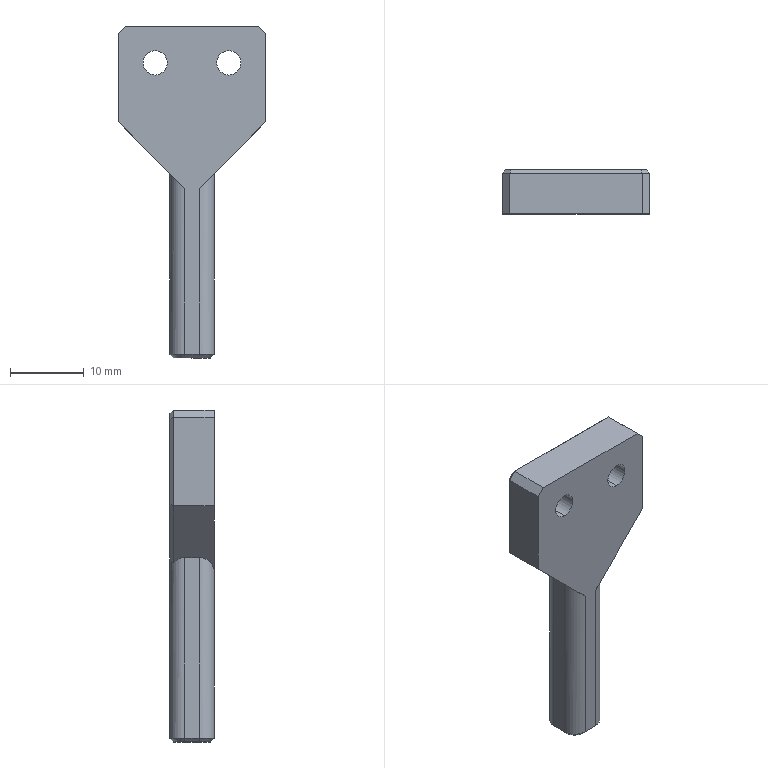Component | SolidWorks | GripperJaw3-1 | 1 solid | 35 faces | box 20 x 6 x 45 mm | volume 2802 mm3 | plane 23 | cylinder 8 | cone 4 | commonest cylinder face diameters 3.3 x4 4 x4
STEP:
#1=COLOUR_RGB('',0.7922,0.8196,0.9333);
#2=FILL_AREA_STYLE_COLOUR('',#1);
#3=FILL_AREA_STYLE('',(#2));
#4=SURFACE_STYLE_FILL_AREA(#3);
#5=SURFACE_SIDE_STYLE('',(#4));
#6=SURFACE_STYLE_USAGE(.BOTH.,#5);
#7=PRESENTATION_STYLE_ASSIGNMENT((#6));
#8=CARTESIAN_POINT('',(-1.976,-2.415,3.085));
#9=VERTEX_POINT('',#8);
#10=CARTESIAN_POINT('',(-1.976,-2.415,2.956));
#11=VERTEX_POINT('',#10);
#12=CARTESIAN_POINT('',(-1.976,-2.415,3.02));
#13=DIRECTION('',(-0.,1.,-0.));
#14=DIRECTION('',(0.,0.,-1.));
#15=AXIS2_PLACEMENT_3D('',#12,#13,#14);
#16=CIRCLE('',#15,0.06496);
#17=EDGE_CURVE('',#9,#11,#16,.T.);
#18=ORIENTED_EDGE('',*,*,#17,.F.);
#19=CARTESIAN_POINT('',(-1.976,-2.179,3.085));
#20=VERTEX_POINT('',#19);
#21=CARTESIAN_POINT('',(-1.976,-2.179,3.085));
#22=DIRECTION('',(-0.,1.,-0.));
#23=VECTOR('',#22,39.37);
#24=LINE('',#21,#23);
#25=EDGE_CURVE('',#9,#20,#24,.T.);
#26=ORIENTED_EDGE('',*,*,#25,.T.);
#27=CARTESIAN_POINT('',(-1.976,-2.179,2.956));
#28=VERTEX_POINT('',#27);
#29=CARTESIAN_POINT('',(-1.976,-2.179,3.02));
#30=DIRECTION('',(-0.,1.,-0.));
#31=DIRECTION('',(0.,0.,-1.));
#32=AXIS2_PLACEMENT_3D('',#29,#30,#31);
#33=CIRCLE('',#32,0.06496);
#34=EDGE_CURVE('',#20,#28,#33,.T.);
#35=ORIENTED_EDGE('',*,*,#34,.T.);
#36=CARTESIAN_POINT('',(-1.976,-2.179,2.956));
#37=DIRECTION('',(-0.,1.,-0.));
#38=VECTOR('',#37,39.37);
#39=LINE('',#36,#38);
#40=EDGE_CURVE('',#11,#28,#39,.T.);
#41=ORIENTED_EDGE('',*,*,#40,.F.);
#42=EDGE_LOOP('',(#18,#26,#35,#41));
#43=FACE_OUTER_BOUND('',#42,.T.);
#44=CARTESIAN_POINT('',(-1.976,-2.179,3.02));
#45=DIRECTION('',(-0.,1.,-0.));
#46=DIRECTION('',(0.,0.,-1.));
#47=AXIS2_PLACEMENT_3D('',#44,#45,#46);
#48=CYLINDRICAL_SURFACE('',#47,0.06496);
#49=ADVANCED_FACE('',(#43),#48,.F.);
#50=CARTESIAN_POINT('',(-1.582,-2.415,3.085));
#51=VERTEX_POINT('',#50);
#52=CARTESIAN_POINT('',(-1.582,-2.415,2.956));
#53=VERTEX_POINT('',#52);
#54=CARTESIAN_POINT('',(-1.582,-2.415,3.02));
#55=DIRECTION('',(-0.,1.,-0.));
#56=DIRECTION('',(0.,0.,-1.));
#57=AXIS2_PLACEMENT_3D('',#54,#55,#56);
#58=CIRCLE('',#57,0.06496);
#59=EDGE_CURVE('',#51,#53,#58,.T.);
#60=ORIENTED_EDGE('',*,*,#59,.F.);
#61=CARTESIAN_POINT('',(-1.582,-2.179,3.085));
#62=VERTEX_POINT('',#61);
#63=CARTESIAN_POINT('',(-1.582,-2.179,3.085));
#64=DIRECTION('',(-0.,1.,-0.));
#65=VECTOR('',#64,39.37);
#66=LINE('',#63,#65);
#67=EDGE_CURVE('',#51,#62,#66,.T.);
#68=ORIENTED_EDGE('',*,*,#67,.T.);
#69=CARTESIAN_POINT('',(-1.582,-2.179,2.956));
#70=VERTEX_POINT('',#69);
#71=CARTESIAN_POINT('',(-1.582,-2.179,3.02));
#72=DIRECTION('',(-0.,1.,-0.));
#73=DIRECTION('',(0.,0.,-1.));
#74=AXIS2_PLACEMENT_3D('',#71,#72,#73);
#75=CIRCLE('',#74,0.06496);
#76=EDGE_CURVE('',#62,#70,#75,.T.);
#77=ORIENTED_EDGE('',*,*,#76,.T.);
#78=CARTESIAN_POINT('',(-1.582,-2.179,2.956));
#79=DIRECTION('',(-0.,1.,-0.));
#80=VECTOR('',#79,39.37);
#81=LINE('',#78,#80);
#82=EDGE_CURVE('',#53,#70,#81,.T.);
#83=ORIENTED_EDGE('',*,*,#82,.F.);
#84=EDGE_LOOP('',(#60,#68,#77,#83));
#85=FACE_OUTER_BOUND('',#84,.T.);
#86=CARTESIAN_POINT('',(-1.582,-2.179,3.02));
#87=DIRECTION('',(-0.,1.,-0.));
#88=DIRECTION('',(0.,0.,-1.));
#89=AXIS2_PLACEMENT_3D('',#86,#87,#88);
#90=CYLINDRICAL_SURFACE('',#89,0.06496);
#91=ADVANCED_FACE('',(#85),#90,.F.);
#92=CARTESIAN_POINT('',(-1.681,-2.336,1.446));
#93=VERTEX_POINT('',#92);
#94=CARTESIAN_POINT('',(-1.74,-2.395,1.446));
#95=VERTEX_POINT('',#94);
#96=CARTESIAN_POINT('',(-1.74,-2.336,1.446));
#97=DIRECTION('',(-0.,0.,-1.));
#98=DIRECTION('',(1.,0.,0.));
#99=AXIS2_PLACEMENT_3D('',#96,#97,#98);
#100=CIRCLE('',#99,0.05906);
#101=EDGE_CURVE('',#93,#95,#100,.T.);
#102=ORIENTED_EDGE('',*,*,#101,.T.);
#103=CARTESIAN_POINT('',(-1.818,-2.395,1.446));
#104=VERTEX_POINT('',#103);
#105=CARTESIAN_POINT('',(-2.173,-2.395,1.446));
#106=DIRECTION('',(-1.,0.,0.));
#107=VECTOR('',#106,39.37);
#108=LINE('',#105,#107);
#109=EDGE_CURVE('',#95,#104,#108,.T.);
#110=ORIENTED_EDGE('',*,*,#109,.T.);
#111=CARTESIAN_POINT('',(-1.877,-2.336,1.446));
#112=VERTEX_POINT('',#111);
#113=CARTESIAN_POINT('',(-1.818,-2.336,1.446));
#114=DIRECTION('',(-0.,0.,-1.));
#115=DIRECTION('',(1.,0.,0.));
#116=AXIS2_PLACEMENT_3D('',#113,#114,#115);
#117=CIRCLE('',#116,0.05906);
#118=EDGE_CURVE('',#104,#112,#117,.T.);
#119=ORIENTED_EDGE('',*,*,#118,.T.);
#120=CARTESIAN_POINT('',(-1.877,-2.258,1.446));
#121=VERTEX_POINT('',#120);
#122=CARTESIAN_POINT('',(-1.877,-2.179,1.446));
#123=DIRECTION('',(-0.,1.,-0.));
#124=VECTOR('',#123,39.37);
#125=LINE('',#122,#124);
#126=EDGE_CURVE('',#112,#121,#125,.T.);
#127=ORIENTED_EDGE('',*,*,#126,.T.);
#128=CARTESIAN_POINT('',(-1.818,-2.199,1.446));
#129=VERTEX_POINT('',#128);
#130=CARTESIAN_POINT('',(-1.818,-2.258,1.446));
#131=DIRECTION('',(-0.,0.,-1.));
#132=DIRECTION('',(1.,0.,0.));
#133=AXIS2_PLACEMENT_3D('',#130,#131,#132);
#134=CIRCLE('',#133,0.05906);
#135=EDGE_CURVE('',#121,#129,#134,.T.);
#136=ORIENTED_EDGE('',*,*,#135,.T.);
#137=CARTESIAN_POINT('',(-1.74,-2.199,1.446));
#138=VERTEX_POINT('',#137);
#139=CARTESIAN_POINT('',(-1.74,-2.199,1.446));
#140=DIRECTION('',(1.,-0.,-0.));
#141=VECTOR('',#140,39.37);
#142=LINE('',#139,#141);
#143=EDGE_CURVE('',#129,#138,#142,.T.);
#144=ORIENTED_EDGE('',*,*,#143,.T.);
#145=CARTESIAN_POINT('',(-1.681,-2.258,1.446));
#146=VERTEX_POINT('',#145);
#147=CARTESIAN_POINT('',(-1.74,-2.258,1.446));
#148=DIRECTION('',(-0.,0.,-1.));
#149=DIRECTION('',(1.,0.,0.));
#150=AXIS2_PLACEMENT_3D('',#147,#148,#149);
#151=CIRCLE('',#150,0.05906);
#152=EDGE_CURVE('',#138,#146,#151,.T.);
#153=ORIENTED_EDGE('',*,*,#152,.T.);
#154=CARTESIAN_POINT('',(-1.681,-2.179,1.446));
#155=DIRECTION('',(0.,-1.,0.));
#156=VECTOR('',#155,39.37);
#157=LINE('',#154,#156);
#158=EDGE_CURVE('',#146,#93,#157,.T.);
#159=ORIENTED_EDGE('',*,*,#158,.T.);
#160=EDGE_LOOP('',(#102,#110,#119,#127,#136,#144,#153,#159));
#161=FACE_OUTER_BOUND('',#160,.T.);
#162=CARTESIAN_POINT('',(-2.173,-2.179,1.446));
#163=DIRECTION('',(0.,-0.,1.));
#164=DIRECTION('',(1.,-0.,-0.));
#165=AXIS2_PLACEMENT_3D('',#162,#163,#164);
#166=PLANE('',#165);
#167=ADVANCED_FACE('',(#161),#166,.F.);
#168=CARTESIAN_POINT('',(-2.173,-2.415,3.178));
#169=VERTEX_POINT('',#168);
#170=CARTESIAN_POINT('',(-2.173,-2.199,3.178));
#171=VERTEX_POINT('',#170);
#172=CARTESIAN_POINT('',(-2.173,-2.179,3.178));
#173=DIRECTION('',(-0.,1.,-0.));
#174=VECTOR('',#173,39.37);
#175=LINE('',#172,#174);
#176=EDGE_CURVE('',#169,#171,#175,.T.);
#177=ORIENTED_EDGE('',*,*,#176,.T.);
#178=CARTESIAN_POINT('',(-2.173,-2.199,2.706));
#179=VERTEX_POINT('',#178);
#180=CARTESIAN_POINT('',(-2.173,-2.199,2.706));
#181=DIRECTION('',(-0.,0.,-1.));
#182=VECTOR('',#181,39.37);
#183=LINE('',#180,#182);
#184=EDGE_CURVE('',#171,#179,#183,.T.);
#185=ORIENTED_EDGE('',*,*,#184,.T.);
#186=CARTESIAN_POINT('',(-2.173,-2.415,2.706));
#187=VERTEX_POINT('',#186);
#188=CARTESIAN_POINT('',(-2.173,-2.179,2.706));
#189=DIRECTION('',(0.,-1.,0.));
#190=VECTOR('',#189,39.37);
#191=LINE('',#188,#190);
#192=EDGE_CURVE('',#179,#187,#191,.T.);
#193=ORIENTED_EDGE('',*,*,#192,.T.);
#194=CARTESIAN_POINT('',(-2.173,-2.415,3.217));
#195=DIRECTION('',(0.,-0.,1.));
#196=VECTOR('',#195,39.37);
#197=LINE('',#194,#196);
#198=EDGE_CURVE('',#187,#169,#197,.T.);
#199=ORIENTED_EDGE('',*,*,#198,.T.);
#200=EDGE_LOOP('',(#177,#185,#193,#199));
#201=FACE_OUTER_BOUND('',#200,.T.);
#202=CARTESIAN_POINT('',(-2.173,-2.179,3.217));
#203=DIRECTION('',(1.,0.,-0.));
#204=DIRECTION('',(0.,-1.,0.));
#205=AXIS2_PLACEMENT_3D('',#202,#203,#204);
#206=PLANE('',#205);
#207=ADVANCED_FACE('',(#201),#206,.F.);
#208=CARTESIAN_POINT('',(-1.425,-2.415,3.217));
#209=VERTEX_POINT('',#208);
#210=CARTESIAN_POINT('',(-1.425,-2.199,3.217));
#211=VERTEX_POINT('',#210);
#212=CARTESIAN_POINT('',(-1.425,-2.179,3.217));
#213=DIRECTION('',(-0.,1.,-0.));
#214=VECTOR('',#213,39.37);
#215=LINE('',#212,#214);
#216=EDGE_CURVE('',#209,#211,#215,.T.);
#217=ORIENTED_EDGE('',*,*,#216,.T.);
#218=CARTESIAN_POINT('',(-2.133,-2.199,3.217));
#219=VERTEX_POINT('',#218);
#220=CARTESIAN_POINT('',(-2.133,-2.199,3.217));
#221=DIRECTION('',(-1.,0.,0.));
#222=VECTOR('',#221,39.37);
#223=LINE('',#220,#222);
#224=EDGE_CURVE('',#211,#219,#223,.T.);
#225=ORIENTED_EDGE('',*,*,#224,.T.);
#226=CARTESIAN_POINT('',(-2.133,-2.415,3.217));
#227=VERTEX_POINT('',#226);
#228=CARTESIAN_POINT('',(-2.133,-2.179,3.217));
#229=DIRECTION('',(0.,-1.,0.));
#230=VECTOR('',#229,39.37);
#231=LINE('',#228,#230);
#232=EDGE_CURVE('',#219,#227,#231,.T.);
#233=ORIENTED_EDGE('',*,*,#232,.T.);
#234=CARTESIAN_POINT('',(-2.173,-2.415,3.217));
#235=DIRECTION('',(1.,-0.,-0.));
#236=VECTOR('',#235,39.37);
#237=LINE('',#234,#236);
#238=EDGE_CURVE('',#227,#209,#237,.T.);
#239=ORIENTED_EDGE('',*,*,#238,.T.);
#240=EDGE_LOOP('',(#217,#225,#233,#239));
#241=FACE_OUTER_BOUND('',#240,.T.);
#242=CARTESIAN_POINT('',(-2.173,-2.179,3.217));
#243=DIRECTION('',(-0.,0.,-1.));
#244=DIRECTION('',(-1.,0.,0.));
#245=AXIS2_PLACEMENT_3D('',#242,#243,#244);
#246=PLANE('',#245);
#247=ADVANCED_FACE('',(#241),#246,.F.);
#248=CARTESIAN_POINT('',(-1.385,-2.415,2.706));
#249=VERTEX_POINT('',#248);
#250=CARTESIAN_POINT('',(-1.385,-2.199,2.706));
#251=VERTEX_POINT('',#250);
#252=CARTESIAN_POINT('',(-1.385,-2.179,2.706));
#253=DIRECTION('',(-0.,1.,-0.));
#254=VECTOR('',#253,39.37);
#255=LINE('',#252,#254);
#256=EDGE_CURVE('',#249,#251,#255,.T.);
#257=ORIENTED_EDGE('',*,*,#256,.T.);
#258=CARTESIAN_POINT('',(-1.385,-2.199,3.178));
#259=VERTEX_POINT('',#258);
#260=CARTESIAN_POINT('',(-1.385,-2.199,3.178));
#261=DIRECTION('',(0.,-0.,1.));
#262=VECTOR('',#261,39.37);
#263=LINE('',#260,#262);
#264=EDGE_CURVE('',#251,#259,#263,.T.);
#265=ORIENTED_EDGE('',*,*,#264,.T.);
#266=CARTESIAN_POINT('',(-1.385,-2.415,3.178));
#267=VERTEX_POINT('',#266);
#268=CARTESIAN_POINT('',(-1.385,-2.179,3.178));
#269=DIRECTION('',(0.,-1.,0.));
#270=VECTOR('',#269,39.37);
#271=LINE('',#268,#270);
#272=EDGE_CURVE('',#259,#267,#271,.T.);
#273=ORIENTED_EDGE('',*,*,#272,.T.);
#274=CARTESIAN_POINT('',(-1.385,-2.415,3.217));
#275=DIRECTION('',(-0.,0.,-1.));
#276=VECTOR('',#275,39.37);
#277=LINE('',#274,#276);
#278=EDGE_CURVE('',#267,#249,#277,.T.);
#279=ORIENTED_EDGE('',*,*,#278,.T.);
#280=EDGE_LOOP('',(#257,#265,#273,#279));
#281=FACE_OUTER_BOUND('',#280,.T.);
#282=CARTESIAN_POINT('',(-1.385,-2.179,3.217));
#283=DIRECTION('',(-1.,-0.,0.));
#284=DIRECTION('',(-0.,1.,-0.));
#285=AXIS2_PLACEMENT_3D('',#282,#283,#284);
#286=PLANE('',#285);
#287=ADVANCED_FACE('',(#281),#286,.F.);
#288=CARTESIAN_POINT('',(-1.74,-2.179,2.379));
#289=VERTEX_POINT('',#288);
#290=CARTESIAN_POINT('',(-1.74,-2.179,1.465));
#291=VERTEX_POINT('',#290);
#292=CARTESIAN_POINT('',(-1.74,-2.179,1.446));
#293=DIRECTION('',(-0.,0.,-1.));
#294=VECTOR('',#293,39.37);
#295=LINE('',#292,#294);
#296=EDGE_CURVE('',#289,#291,#295,.T.);
#297=ORIENTED_EDGE('',*,*,#296,.T.);
#298=CARTESIAN_POINT('',(-1.818,-2.179,1.465));
#299=VERTEX_POINT('',#298);
#300=CARTESIAN_POINT('',(-1.818,-2.179,1.465));
#301=DIRECTION('',(-1.,0.,0.));
#302=VECTOR('',#301,39.37);
#303=LINE('',#300,#302);
#304=EDGE_CURVE('',#291,#299,#303,.T.);
#305=ORIENTED_EDGE('',*,*,#304,.T.);
#306=CARTESIAN_POINT('',(-1.818,-2.179,2.379));
#307=VERTEX_POINT('',#306);
#308=CARTESIAN_POINT('',(-1.818,-2.179,2.43));
#309=DIRECTION('',(0.,-0.,1.));
#310=VECTOR('',#309,39.37);
#311=LINE('',#308,#310);
#312=EDGE_CURVE('',#299,#307,#311,.T.);
#313=ORIENTED_EDGE('',*,*,#312,.T.);
#314=CARTESIAN_POINT('',(-2.153,-2.179,2.714));
#315=VERTEX_POINT('',#314);
#316=CARTESIAN_POINT('',(-2.159,-2.179,2.719));
#317=DIRECTION('',(-0.7071,-0.,0.7071));
#318=VECTOR('',#317,39.37);
#319=LINE('',#316,#318);
#320=EDGE_CURVE('',#307,#315,#319,.T.);
#321=ORIENTED_EDGE('',*,*,#320,.T.);
#322=CARTESIAN_POINT('',(-2.153,-2.179,3.17));
#323=VERTEX_POINT('',#322);
#324=CARTESIAN_POINT('',(-2.153,-2.179,3.178));
#325=DIRECTION('',(0.,-0.,1.));
#326=VECTOR('',#325,39.37);
#327=LINE('',#324,#326);
#328=EDGE_CURVE('',#315,#323,#327,.T.);
#329=ORIENTED_EDGE('',*,*,#328,.T.);
#330=CARTESIAN_POINT('',(-2.125,-2.179,3.198));
#331=VERTEX_POINT('',#330);
#332=CARTESIAN_POINT('',(-2.385,-2.179,2.938));
#333=DIRECTION('',(0.7071,-0.,0.7071));
#334=VECTOR('',#333,39.37);
#335=LINE('',#332,#334);
#336=EDGE_CURVE('',#323,#331,#335,.T.);
#337=ORIENTED_EDGE('',*,*,#336,.T.);
#338=CARTESIAN_POINT('',(-1.433,-2.179,3.198));
#339=VERTEX_POINT('',#338);
#340=CARTESIAN_POINT('',(-1.425,-2.179,3.198));
#341=DIRECTION('',(1.,-0.,-0.));
#342=VECTOR('',#341,39.37);
#343=LINE('',#340,#342);
#344=EDGE_CURVE('',#331,#339,#343,.T.);
#345=ORIENTED_EDGE('',*,*,#344,.T.);
#346=CARTESIAN_POINT('',(-1.405,-2.179,3.17));
#347=VERTEX_POINT('',#346);
#348=CARTESIAN_POINT('',(-1.173,-2.179,2.938));
#349=DIRECTION('',(0.7071,0.,-0.7071));
#350=VECTOR('',#349,39.37);
#351=LINE('',#348,#350);
#352=EDGE_CURVE('',#339,#347,#351,.T.);
#353=ORIENTED_EDGE('',*,*,#352,.T.);
#354=CARTESIAN_POINT('',(-1.405,-2.179,2.714));
#355=VERTEX_POINT('',#354);
#356=CARTESIAN_POINT('',(-1.405,-2.179,2.706));
#357=DIRECTION('',(-0.,0.,-1.));
#358=VECTOR('',#357,39.37);
#359=LINE('',#356,#358);
#360=EDGE_CURVE('',#347,#355,#359,.T.);
#361=ORIENTED_EDGE('',*,*,#360,.T.);
#362=CARTESIAN_POINT('',(-1.754,-2.179,2.365));
#363=DIRECTION('',(-0.7071,0.,-0.7071));
#364=VECTOR('',#363,39.37);
#365=LINE('',#362,#364);
#366=EDGE_CURVE('',#355,#289,#365,.T.);
#367=ORIENTED_EDGE('',*,*,#366,.T.);
#368=EDGE_LOOP('',(#297,#305,#313,#321,#329,#337,#345,#353,#361,#367));
#369=FACE_OUTER_BOUND('',#368,.T.);
#370=CARTESIAN_POINT('',(-1.976,-2.179,3.02));
#371=DIRECTION('',(-0.,1.,-0.));
#372=DIRECTION('',(0.,0.,-1.));
#373=AXIS2_PLACEMENT_3D('',#370,#371,#372);
#374=CIRCLE('',#373,0.06496);
#375=EDGE_CURVE('',#28,#20,#374,.T.);
#376=ORIENTED_EDGE('',*,*,#375,.F.);
#377=ORIENTED_EDGE('',*,*,#34,.F.);
#378=EDGE_LOOP('',(#376,#377));
#379=FACE_BOUND('',#378,.T.);
#380=CARTESIAN_POINT('',(-1.582,-2.179,3.02));
#381=DIRECTION('',(-0.,1.,-0.));
#382=DIRECTION('',(0.,0.,-1.));
#383=AXIS2_PLACEMENT_3D('',#380,#381,#382);
#384=CIRCLE('',#383,0.06496);
#385=EDGE_CURVE('',#70,#62,#384,.T.);
#386=ORIENTED_EDGE('',*,*,#385,.F.);
#387=ORIENTED_EDGE('',*,*,#76,.F.);
#388=EDGE_LOOP('',(#386,#387));
#389=FACE_BOUND('',#388,.T.);
#390=CARTESIAN_POINT('',(-1.779,-2.179,2.331));
#391=DIRECTION('',(-0.,1.,0.));
#392=DIRECTION('',(-0.,0.,-1.));
#393=AXIS2_PLACEMENT_3D('',#390,#391,#392);
#394=PLANE('',#393);
#395=ADVANCED_FACE('',(#369,#379,#389),#394,.T.);
#396=CARTESIAN_POINT('',(-1.976,-2.415,3.02));
#397=DIRECTION('',(-0.,1.,-0.));
#398=DIRECTION('',(0.,0.,-1.));
#399=AXIS2_PLACEMENT_3D('',#396,#397,#398);
#400=CIRCLE('',#399,0.06496);
#401=EDGE_CURVE('',#11,#9,#400,.T.);
#402=ORIENTED_EDGE('',*,*,#401,.T.);
#403=ORIENTED_EDGE('',*,*,#17,.T.);
#404=EDGE_LOOP('',(#402,#403));
#405=FACE_BOUND('',#404,.T.);
#406=CARTESIAN_POINT('',(-1.582,-2.415,3.02));
#407=DIRECTION('',(-0.,1.,-0.));
#408=DIRECTION('',(0.,0.,-1.));
#409=AXIS2_PLACEMENT_3D('',#406,#407,#408);
#410=CIRCLE('',#409,0.06496);
#411=EDGE_CURVE('',#53,#51,#410,.T.);
#412=ORIENTED_EDGE('',*,*,#411,.T.);
#413=ORIENTED_EDGE('',*,*,#59,.T.);
#414=EDGE_LOOP('',(#412,#413));
#415=FACE_BOUND('',#414,.T.);
#416=CARTESIAN_POINT('',(-1.818,-2.415,2.351));
#417=VERTEX_POINT('',#416);
#418=CARTESIAN_POINT('',(-1.818,-2.415,1.465));
#419=VERTEX_POINT('',#418);
#420=CARTESIAN_POINT('',(-1.818,-2.415,2.331));
#421=DIRECTION('',(-0.,0.,-1.));
#422=VECTOR('',#421,39.37);
#423=LINE('',#420,#422);
#424=EDGE_CURVE('',#417,#419,#423,.T.);
#425=ORIENTED_EDGE('',*,*,#424,.T.);
#426=CARTESIAN_POINT('',(-1.74,-2.415,1.465));
#427=VERTEX_POINT('',#426);
#428=CARTESIAN_POINT('',(-1.779,-2.415,1.465));
#429=DIRECTION('',(1.,-0.,-0.));
#430=VECTOR('',#429,39.37);
#431=LINE('',#428,#430);
#432=EDGE_CURVE('',#419,#427,#431,.T.);
#433=ORIENTED_EDGE('',*,*,#432,.T.);
#434=CARTESIAN_POINT('',(-1.74,-2.415,2.351));
#435=VERTEX_POINT('',#434);
#436=CARTESIAN_POINT('',(-1.74,-2.415,2.331));
#437=DIRECTION('',(0.,-0.,1.));
#438=VECTOR('',#437,39.37);
#439=LINE('',#436,#438);
#440=EDGE_CURVE('',#427,#435,#439,.T.);
#441=ORIENTED_EDGE('',*,*,#440,.T.);
#442=CARTESIAN_POINT('',(-1.769,-2.415,2.322));
#443=DIRECTION('',(0.7071,-0.,0.7071));
#444=VECTOR('',#443,39.37);
#445=LINE('',#442,#444);
#446=EDGE_CURVE('',#435,#249,#445,.T.);
#447=ORIENTED_EDGE('',*,*,#446,.T.);
#448=ORIENTED_EDGE('',*,*,#278,.F.);
#449=CARTESIAN_POINT('',(-1.385,-2.415,3.178));
#450=DIRECTION('',(-0.7071,-0.,0.7071));
#451=VECTOR('',#450,39.37);
#452=LINE('',#449,#451);
#453=EDGE_CURVE('',#267,#209,#452,.T.);
#454=ORIENTED_EDGE('',*,*,#453,.T.);
#455=ORIENTED_EDGE('',*,*,#238,.F.);
#456=CARTESIAN_POINT('',(-2.133,-2.415,3.217));
#457=DIRECTION('',(-0.7071,0.,-0.7071));
#458=VECTOR('',#457,39.37);
#459=LINE('',#456,#458);
#460=EDGE_CURVE('',#227,#169,#459,.T.);
#461=ORIENTED_EDGE('',*,*,#460,.T.);
#462=ORIENTED_EDGE('',*,*,#198,.F.);
#463=CARTESIAN_POINT('',(-1.789,-2.415,2.322));
#464=DIRECTION('',(0.7071,0.,-0.7071));
#465=VECTOR('',#464,39.37);
#466=LINE('',#463,#465);
#467=EDGE_CURVE('',#187,#417,#466,.T.);
#468=ORIENTED_EDGE('',*,*,#467,.T.);
#469=EDGE_LOOP('',(#425,#433,#441,#447,#448,#454,#455,#461,#462,#468));
#470=FACE_OUTER_BOUND('',#469,.T.);
#471=CARTESIAN_POINT('',(-1.779,-2.415,2.331));
#472=DIRECTION('',(-0.,1.,0.));
#473=DIRECTION('',(-0.,0.,-1.));
#474=AXIS2_PLACEMENT_3D('',#471,#472,#473);
#475=PLANE('',#474);
#476=ADVANCED_FACE('',(#405,#415,#470),#475,.F.);
#477=ORIENTED_EDGE('',*,*,#67,.F.);
#478=ORIENTED_EDGE('',*,*,#411,.F.);
#479=ORIENTED_EDGE('',*,*,#82,.T.);
#480=ORIENTED_EDGE('',*,*,#385,.T.);
#481=EDGE_LOOP('',(#477,#478,#479,#480));
#482=FACE_OUTER_BOUND('',#481,.T.);
#483=CARTESIAN_POINT('',(-1.582,-2.179,3.02));
#484=DIRECTION('',(-0.,1.,-0.));
#485=DIRECTION('',(0.,0.,-1.));
#486=AXIS2_PLACEMENT_3D('',#483,#484,#485);
#487=CYLINDRICAL_SURFACE('',#486,0.06496);
#488=ADVANCED_FACE('',(#482),#487,.F.);
#489=ORIENTED_EDGE('',*,*,#25,.F.);
#490=ORIENTED_EDGE('',*,*,#401,.F.);
#491=ORIENTED_EDGE('',*,*,#40,.T.);
#492=ORIENTED_EDGE('',*,*,#375,.T.);
#493=EDGE_LOOP('',(#489,#490,#491,#492));
#494=FACE_OUTER_BOUND('',#493,.T.);
#495=CARTESIAN_POINT('',(-1.976,-2.179,3.02));
#496=DIRECTION('',(-0.,1.,-0.));
#497=DIRECTION('',(0.,0.,-1.));
#498=AXIS2_PLACEMENT_3D('',#495,#496,#497);
#499=CYLINDRICAL_SURFACE('',#498,0.06496);
#500=ADVANCED_FACE('',(#494),#499,.F.);
#501=CARTESIAN_POINT('',(-1.661,-2.336,2.43));
#502=VERTEX_POINT('',#501);
#503=CARTESIAN_POINT('',(-1.661,-2.336,1.465));
#504=VERTEX_POINT('',#503);
#505=CARTESIAN_POINT('',(-1.661,-2.336,1.446));
#506=DIRECTION('',(-0.,0.,-1.));
#507=VECTOR('',#506,39.37);
#508=LINE('',#505,#507);
#509=EDGE_CURVE('',#502,#504,#508,.T.);
#510=ORIENTED_EDGE('',*,*,#509,.T.);
#511=CARTESIAN_POINT('',(-1.661,-2.258,1.465));
#512=VERTEX_POINT('',#511);
#513=CARTESIAN_POINT('',(-1.661,-2.415,1.465));
#514=DIRECTION('',(-0.,1.,-0.));
#515=VECTOR('',#514,39.37);
#516=LINE('',#513,#515);
#517=EDGE_CURVE('',#504,#512,#516,.T.);
#518=ORIENTED_EDGE('',*,*,#517,.T.);
#519=CARTESIAN_POINT('',(-1.661,-2.258,2.43));
#520=VERTEX_POINT('',#519);
#521=CARTESIAN_POINT('',(-1.661,-2.258,2.43));
#522=DIRECTION('',(0.,-0.,1.));
#523=VECTOR('',#522,39.37);
#524=LINE('',#521,#523);
#525=EDGE_CURVE('',#512,#520,#524,.T.);
#526=ORIENTED_EDGE('',*,*,#525,.T.);
#527=CARTESIAN_POINT('',(-1.661,-2.415,2.43));
#528=DIRECTION('',(0.,-1.,0.));
#529=VECTOR('',#528,39.37);
#530=LINE('',#527,#529);
#531=EDGE_CURVE('',#520,#502,#530,.T.);
#532=ORIENTED_EDGE('',*,*,#531,.T.);
#533=EDGE_LOOP('',(#510,#518,#526,#532));
#534=FACE_OUTER_BOUND('',#533,.T.);
#535=CARTESIAN_POINT('',(-1.661,-2.415,1.446));
#536=DIRECTION('',(-1.,0.,0.));
#537=DIRECTION('',(0.,-0.,1.));
#538=AXIS2_PLACEMENT_3D('',#535,#536,#537);
#539=PLANE('',#538);
#540=ADVANCED_FACE('',(#534),#539,.F.);
#541=CARTESIAN_POINT('',(-1.897,-2.258,2.43));
#542=VERTEX_POINT('',#541);
#543=CARTESIAN_POINT('',(-1.897,-2.258,1.465));
#544=VERTEX_POINT('',#543);
#545=CARTESIAN_POINT('',(-1.897,-2.258,1.446));
#546=DIRECTION('',(-0.,0.,-1.));
#547=VECTOR('',#546,39.37);
#548=LINE('',#545,#547);
#549=EDGE_CURVE('',#542,#544,#548,.T.);
#550=ORIENTED_EDGE('',*,*,#549,.T.);
#551=CARTESIAN_POINT('',(-1.897,-2.336,1.465));
#552=VERTEX_POINT('',#551);
#553=CARTESIAN_POINT('',(-1.897,-2.415,1.465));
#554=DIRECTION('',(0.,-1.,0.));
#555=VECTOR('',#554,39.37);
#556=LINE('',#553,#555);
#557=EDGE_CURVE('',#544,#552,#556,.T.);
#558=ORIENTED_EDGE('',*,*,#557,.T.);
#559=CARTESIAN_POINT('',(-1.897,-2.336,2.43));
#560=VERTEX_POINT('',#559);
#561=CARTESIAN_POINT('',(-1.897,-2.336,1.446));
#562=DIRECTION('',(0.,-0.,1.));
#563=VECTOR('',#562,39.37);
#564=LINE('',#561,#563);
#565=EDGE_CURVE('',#552,#560,#564,.T.);
#566=ORIENTED_EDGE('',*,*,#565,.T.);
#567=CARTESIAN_POINT('',(-1.897,-2.179,2.43));
#568=DIRECTION('',(-0.,1.,-0.));
#569=VECTOR('',#568,39.37);
#570=LINE('',#567,#569);
#571=EDGE_CURVE('',#560,#542,#570,.T.);
#572=ORIENTED_EDGE('',*,*,#571,.T.);
#573=EDGE_LOOP('',(#550,#558,#566,#572));
#574=FACE_OUTER_BOUND('',#573,.T.);
#575=CARTESIAN_POINT('',(-1.897,-2.415,1.446));
#576=DIRECTION('',(1.,-0.,-0.));
#577=DIRECTION('',(-0.,0.,-1.));
#578=AXIS2_PLACEMENT_3D('',#575,#576,#577);
#579=PLANE('',#578);
#580=ADVANCED_FACE('',(#574),#579,.F.);
#581=CARTESIAN_POINT('',(-1.688,-2.199,2.403));
#582=VERTEX_POINT('',#581);
#583=CARTESIAN_POINT('',(-1.661,-2.258,2.43));
#584=CARTESIAN_POINT('',(-1.661,-2.235,2.43));
#585=CARTESIAN_POINT('',(-1.67,-2.214,2.42));
#586=CARTESIAN_POINT('',(-1.688,-2.199,2.403));
#587=(BOUNDED_CURVE()B_SPLINE_CURVE(3,(#583,#584,#585,#586),.UNSPECIFIED.,.F.,.F.)B_SPLINE_CURVE_WITH_KNOTS((4,4),(3.142,3.99),.UNSPECIFIED.)CURVE()GEOMETRIC_REPRESENTATION_ITEM()RATIONAL_B_SPLINE_CURVE((1.,0.941,0.941,1.))REPRESENTATION_ITEM(''));
#588=EDGE_CURVE('',#520,#582,#587,.T.);
#589=ORIENTED_EDGE('',*,*,#588,.T.);
#590=CARTESIAN_POINT('',(-1.385,-2.199,2.706));
#591=DIRECTION('',(0.7071,-0.,0.7071));
#592=VECTOR('',#591,39.37);
#593=LINE('',#590,#592);
#594=EDGE_CURVE('',#582,#251,#593,.T.);
#595=ORIENTED_EDGE('',*,*,#594,.T.);
#596=ORIENTED_EDGE('',*,*,#256,.F.);
#597=ORIENTED_EDGE('',*,*,#446,.F.);
#598=CARTESIAN_POINT('',(-1.74,-2.415,2.351));
#599=CARTESIAN_POINT('',(-1.694,-2.415,2.397));
#600=CARTESIAN_POINT('',(-1.661,-2.382,2.43));
#601=CARTESIAN_POINT('',(-1.661,-2.336,2.43));
#602=(BOUNDED_CURVE()B_SPLINE_CURVE(3,(#598,#599,#600,#601),.UNSPECIFIED.,.F.,.F.)B_SPLINE_CURVE_WITH_KNOTS((4,4),(4.712,6.283),.UNSPECIFIED.)CURVE()GEOMETRIC_REPRESENTATION_ITEM()RATIONAL_B_SPLINE_CURVE((1.,0.8047,0.8047,1.))REPRESENTATION_ITEM(''));
#603=EDGE_CURVE('',#435,#502,#602,.T.);
#604=ORIENTED_EDGE('',*,*,#603,.T.);
#605=ORIENTED_EDGE('',*,*,#531,.F.);
#606=EDGE_LOOP('',(#589,#595,#596,#597,#604,#605));
#607=FACE_OUTER_BOUND('',#606,.T.);
#608=CARTESIAN_POINT('',(-1.267,-2.415,2.824));
#609=DIRECTION('',(0.7071,-0.,-0.7071));
#610=DIRECTION('',(0.,-1.,0.));
#611=AXIS2_PLACEMENT_3D('',#608,#609,#610);
#612=PLANE('',#611);
#613=ADVANCED_FACE('',(#607),#612,.T.);
#614=ORIENTED_EDGE('',*,*,#192,.F.);
#615=CARTESIAN_POINT('',(-1.871,-2.199,2.403));
#616=VERTEX_POINT('',#615);
#617=CARTESIAN_POINT('',(-1.818,-2.199,2.351));
#618=DIRECTION('',(0.7071,0.,-0.7071));
#619=VECTOR('',#618,39.37);
#620=LINE('',#617,#619);
#621=EDGE_CURVE('',#179,#616,#620,.T.);
#622=ORIENTED_EDGE('',*,*,#621,.T.);
#623=CARTESIAN_POINT('',(-1.871,-2.199,2.403));
#624=CARTESIAN_POINT('',(-1.888,-2.214,2.42));
#625=CARTESIAN_POINT('',(-1.897,-2.235,2.43));
#626=CARTESIAN_POINT('',(-1.897,-2.258,2.43));
#627=(BOUNDED_CURVE()B_SPLINE_CURVE(3,(#623,#624,#625,#626),.UNSPECIFIED.,.F.,.F.)B_SPLINE_CURVE_WITH_KNOTS((4,4),(5.435,6.283),.UNSPECIFIED.)CURVE()GEOMETRIC_REPRESENTATION_ITEM()RATIONAL_B_SPLINE_CURVE((1.,0.941,0.941,1.))REPRESENTATION_ITEM(''));
#628=EDGE_CURVE('',#616,#542,#627,.T.);
#629=ORIENTED_EDGE('',*,*,#628,.T.);
#630=ORIENTED_EDGE('',*,*,#571,.F.);
#631=CARTESIAN_POINT('',(-1.897,-2.336,2.43));
#632=CARTESIAN_POINT('',(-1.897,-2.382,2.43));
#633=CARTESIAN_POINT('',(-1.865,-2.415,2.397));
#634=CARTESIAN_POINT('',(-1.818,-2.415,2.351));
#635=(BOUNDED_CURVE()B_SPLINE_CURVE(3,(#631,#632,#633,#634),.UNSPECIFIED.,.F.,.F.)B_SPLINE_CURVE_WITH_KNOTS((4,4),(3.142,4.712),.UNSPECIFIED.)CURVE()GEOMETRIC_REPRESENTATION_ITEM()RATIONAL_B_SPLINE_CURVE((1.,0.8047,0.8047,1.))REPRESENTATION_ITEM(''));
#636=EDGE_CURVE('',#560,#417,#635,.T.);
#637=ORIENTED_EDGE('',*,*,#636,.T.);
#638=ORIENTED_EDGE('',*,*,#467,.F.);
#639=EDGE_LOOP('',(#614,#622,#629,#630,#637,#638));
#640=FACE_OUTER_BOUND('',#639,.T.);
#641=CARTESIAN_POINT('',(-1.897,-2.415,2.43));
#642=DIRECTION('',(-0.7071,-0.,-0.7071));
#643=DIRECTION('',(0.,-1.,0.));
#644=AXIS2_PLACEMENT_3D('',#641,#642,#643);
#645=PLANE('',#644);
#646=ADVANCED_FACE('',(#640),#645,.T.);
#647=ORIENTED_EDGE('',*,*,#565,.F.);
#648=CARTESIAN_POINT('',(-1.818,-2.336,1.465));
#649=DIRECTION('',(0.,-0.,1.));
#650=DIRECTION('',(0.,1.,0.));
#651=AXIS2_PLACEMENT_3D('',#648,#649,#650);
#652=CIRCLE('',#651,0.07874);
#653=EDGE_CURVE('',#552,#419,#652,.T.);
#654=ORIENTED_EDGE('',*,*,#653,.T.);
#655=ORIENTED_EDGE('',*,*,#424,.F.);
#656=ORIENTED_EDGE('',*,*,#636,.F.);
#657=EDGE_LOOP('',(#647,#654,#655,#656));
#658=FACE_OUTER_BOUND('',#657,.T.);
#659=CARTESIAN_POINT('',(-1.818,-2.336,2.331));
#660=DIRECTION('',(-0.,0.,-1.));
#661=DIRECTION('',(-1.,0.,0.));
#662=AXIS2_PLACEMENT_3D('',#659,#660,#661);
#663=CYLINDRICAL_SURFACE('',#662,0.07874);
#664=ADVANCED_FACE('',(#658),#663,.T.);
#665=ORIENTED_EDGE('',*,*,#440,.F.);
#666=CARTESIAN_POINT('',(-1.74,-2.336,1.465));
#667=DIRECTION('',(0.,-0.,1.));
#668=DIRECTION('',(0.,1.,0.));
#669=AXIS2_PLACEMENT_3D('',#666,#667,#668);
#670=CIRCLE('',#669,0.07874);
#671=EDGE_CURVE('',#427,#504,#670,.T.);
#672=ORIENTED_EDGE('',*,*,#671,.T.);
#673=ORIENTED_EDGE('',*,*,#509,.F.);
#674=ORIENTED_EDGE('',*,*,#603,.F.);
#675=EDGE_LOOP('',(#665,#672,#673,#674));
#676=FACE_OUTER_BOUND('',#675,.T.);
#677=CARTESIAN_POINT('',(-1.74,-2.336,2.331));
#678=DIRECTION('',(0.,-0.,1.));
#679=DIRECTION('',(1.,0.,0.));
#680=AXIS2_PLACEMENT_3D('',#677,#678,#679);
#681=CYLINDRICAL_SURFACE('',#680,0.07874);
#682=ADVANCED_FACE('',(#676),#681,.T.);
#683=ORIENTED_EDGE('',*,*,#312,.F.);
#684=CARTESIAN_POINT('',(-1.818,-2.258,1.465));
#685=DIRECTION('',(0.,-0.,1.));
#686=DIRECTION('',(0.,1.,0.));
#687=AXIS2_PLACEMENT_3D('',#684,#685,#686);
#688=CIRCLE('',#687,0.07874);
#689=EDGE_CURVE('',#299,#544,#688,.T.);
#690=ORIENTED_EDGE('',*,*,#689,.T.);
#691=ORIENTED_EDGE('',*,*,#549,.F.);
#692=ORIENTED_EDGE('',*,*,#628,.F.);
#693=CARTESIAN_POINT('',(-1.871,-2.199,2.403));
#694=CARTESIAN_POINT('',(-1.856,-2.186,2.407));
#695=CARTESIAN_POINT('',(-1.838,-2.179,2.398));
#696=CARTESIAN_POINT('',(-1.818,-2.179,2.379));
#697=(BOUNDED_CURVE()B_SPLINE_CURVE(3,(#693,#694,#695,#696),.UNSPECIFIED.,.F.,.F.)B_SPLINE_CURVE_WITH_KNOTS((4,4),(6.176,6.899),.UNSPECIFIED.)CURVE()GEOMETRIC_REPRESENTATION_ITEM()RATIONAL_B_SPLINE_CURVE((1.,0.9569,0.9569,1.))REPRESENTATION_ITEM(''));
#698=EDGE_CURVE('',#616,#307,#697,.T.);
#699=ORIENTED_EDGE('',*,*,#698,.T.);
#700=EDGE_LOOP('',(#683,#690,#691,#692,#699));
#701=FACE_OUTER_BOUND('',#700,.T.);
#702=CARTESIAN_POINT('',(-1.818,-2.258,1.446));
#703=DIRECTION('',(0.,-0.,1.));
#704=DIRECTION('',(1.,0.,0.));
#705=AXIS2_PLACEMENT_3D('',#702,#703,#704);
#706=CYLINDRICAL_SURFACE('',#705,0.07874);
#707=ADVANCED_FACE('',(#701),#706,.T.);
#708=ORIENTED_EDGE('',*,*,#525,.F.);
#709=CARTESIAN_POINT('',(-1.74,-2.258,1.465));
#710=DIRECTION('',(0.,-0.,1.));
#711=DIRECTION('',(0.,1.,0.));
#712=AXIS2_PLACEMENT_3D('',#709,#710,#711);
#713=CIRCLE('',#712,0.07874);
#714=EDGE_CURVE('',#512,#291,#713,.T.);
#715=ORIENTED_EDGE('',*,*,#714,.T.);
#716=ORIENTED_EDGE('',*,*,#296,.F.);
#717=CARTESIAN_POINT('',(-1.74,-2.179,2.379));
#718=CARTESIAN_POINT('',(-1.72,-2.179,2.398));
#719=CARTESIAN_POINT('',(-1.702,-2.186,2.407));
#720=CARTESIAN_POINT('',(-1.688,-2.199,2.403));
#721=(BOUNDED_CURVE()B_SPLINE_CURVE(3,(#717,#718,#719,#720),.UNSPECIFIED.,.F.,.T.)B_SPLINE_CURVE_WITH_KNOTS((4,4),(2.526,3.249),.UNSPECIFIED.)CURVE()GEOMETRIC_REPRESENTATION_ITEM()RATIONAL_B_SPLINE_CURVE((1.,0.9569,0.9569,1.))REPRESENTATION_ITEM(''));
#722=EDGE_CURVE('',#289,#582,#721,.T.);
#723=ORIENTED_EDGE('',*,*,#722,.T.);
#724=ORIENTED_EDGE('',*,*,#588,.F.);
#725=EDGE_LOOP('',(#708,#715,#716,#723,#724));
#726=FACE_OUTER_BOUND('',#725,.T.);
#727=CARTESIAN_POINT('',(-1.74,-2.258,1.446));
#728=DIRECTION('',(-0.,0.,-1.));
#729=DIRECTION('',(-1.,0.,0.));
#730=AXIS2_PLACEMENT_3D('',#727,#728,#729);
#731=CYLINDRICAL_SURFACE('',#730,0.07874);
#732=ADVANCED_FACE('',(#726),#731,.T.);
#733=ORIENTED_EDGE('',*,*,#272,.F.);
#734=CARTESIAN_POINT('',(-1.385,-2.199,3.178));
#735=DIRECTION('',(-0.7071,-0.,0.7071));
#736=VECTOR('',#735,39.37);
#737=LINE('',#734,#736);
#738=EDGE_CURVE('',#259,#211,#737,.T.);
#739=ORIENTED_EDGE('',*,*,#738,.T.);
#740=ORIENTED_EDGE('',*,*,#216,.F.);
#741=ORIENTED_EDGE('',*,*,#453,.F.);
#742=EDGE_LOOP('',(#733,#739,#740,#741));
#743=FACE_OUTER_BOUND('',#742,.T.);
#744=CARTESIAN_POINT('',(-1.385,-2.179,3.178));
#745=DIRECTION('',(-0.7071,-0.,-0.7071));
#746=DIRECTION('',(0.,-1.,0.));
#747=AXIS2_PLACEMENT_3D('',#744,#745,#746);
#748=PLANE('',#747);
#749=ADVANCED_FACE('',(#743),#748,.F.);
#750=ORIENTED_EDGE('',*,*,#232,.F.);
#751=CARTESIAN_POINT('',(-2.133,-2.199,3.217));
#752=DIRECTION('',(-0.7071,0.,-0.7071));
#753=VECTOR('',#752,39.37);
#754=LINE('',#751,#753);
#755=EDGE_CURVE('',#219,#171,#754,.T.);
#756=ORIENTED_EDGE('',*,*,#755,.T.);
#757=ORIENTED_EDGE('',*,*,#176,.F.);
#758=ORIENTED_EDGE('',*,*,#460,.F.);
#759=EDGE_LOOP('',(#750,#756,#757,#758));
#760=FACE_OUTER_BOUND('',#759,.T.);
#761=CARTESIAN_POINT('',(-2.133,-2.179,3.217));
#762=DIRECTION('',(0.7071,-0.,-0.7071));
#763=DIRECTION('',(0.,-1.,0.));
#764=AXIS2_PLACEMENT_3D('',#761,#762,#763);
#765=PLANE('',#764);
#766=ADVANCED_FACE('',(#760),#765,.F.);
#767=CARTESIAN_POINT('',(-1.818,-2.179,1.465));
#768=DIRECTION('',(-0.,-0.7071,-0.7071));
#769=VECTOR('',#768,39.37);
#770=LINE('',#767,#769);
#771=EDGE_CURVE('',#299,#129,#770,.T.);
#772=ORIENTED_EDGE('',*,*,#771,.F.);
#773=ORIENTED_EDGE('',*,*,#304,.F.);
#774=CARTESIAN_POINT('',(-1.74,-2.199,1.446));
#775=DIRECTION('',(0.,0.7071,0.7071));
#776=VECTOR('',#775,39.37);
#777=LINE('',#774,#776);
#778=EDGE_CURVE('',#138,#291,#777,.T.);
#779=ORIENTED_EDGE('',*,*,#778,.F.);
#780=ORIENTED_EDGE('',*,*,#143,.F.);
#781=EDGE_LOOP('',(#772,#773,#779,#780));
#782=FACE_OUTER_BOUND('',#781,.T.);
#783=CARTESIAN_POINT('',(-1.779,-2.179,1.465));
#784=DIRECTION('',(-0.,0.7071,-0.7071));
#785=DIRECTION('',(1.,-0.,-0.));
#786=AXIS2_PLACEMENT_3D('',#783,#784,#785);
#787=PLANE('',#786);
#788=ADVANCED_FACE('',(#782),#787,.T.);
#789=ORIENTED_EDGE('',*,*,#778,.T.);
#790=ORIENTED_EDGE('',*,*,#714,.F.);
#791=CARTESIAN_POINT('',(-1.681,-2.258,1.446));
#792=DIRECTION('',(0.7071,-0.,0.7071));
#793=VECTOR('',#792,39.37);
#794=LINE('',#791,#793);
#795=EDGE_CURVE('',#146,#512,#794,.T.);
#796=ORIENTED_EDGE('',*,*,#795,.F.);
#797=ORIENTED_EDGE('',*,*,#152,.F.);
#798=EDGE_LOOP('',(#789,#790,#796,#797));
#799=FACE_OUTER_BOUND('',#798,.T.);
#800=CARTESIAN_POINT('',(-1.74,-2.258,1.446));
#801=DIRECTION('',(0.,-0.,1.));
#802=DIRECTION('',(0.,1.,0.));
#803=AXIS2_PLACEMENT_3D('',#800,#801,#802);
#804=CONICAL_SURFACE('',#803,0.05906,0.7854);
#805=ADVANCED_FACE('',(#799),#804,.T.);
#806=ORIENTED_EDGE('',*,*,#771,.T.);
#807=ORIENTED_EDGE('',*,*,#135,.F.);
#808=CARTESIAN_POINT('',(-1.897,-2.258,1.465));
#809=DIRECTION('',(0.7071,0.,-0.7071));
#810=VECTOR('',#809,39.37);
#811=LINE('',#808,#810);
#812=EDGE_CURVE('',#544,#121,#811,.T.);
#813=ORIENTED_EDGE('',*,*,#812,.F.);
#814=ORIENTED_EDGE('',*,*,#689,.F.);
#815=EDGE_LOOP('',(#806,#807,#813,#814));
#816=FACE_OUTER_BOUND('',#815,.T.);
#817=CARTESIAN_POINT('',(-1.818,-2.258,1.446));
#818=DIRECTION('',(0.,-0.,1.));
#819=DIRECTION('',(0.,1.,0.));
#820=AXIS2_PLACEMENT_3D('',#817,#818,#819);
#821=CONICAL_SURFACE('',#820,0.05906,0.7854);
#822=ADVANCED_FACE('',(#816),#821,.T.);
#823=ORIENTED_EDGE('',*,*,#795,.T.);
#824=ORIENTED_EDGE('',*,*,#517,.F.);
#825=CARTESIAN_POINT('',(-1.681,-2.336,1.446));
#826=DIRECTION('',(0.7071,-0.,0.7071));
#827=VECTOR('',#826,39.37);
#828=LINE('',#825,#827);
#829=EDGE_CURVE('',#93,#504,#828,.T.);
#830=ORIENTED_EDGE('',*,*,#829,.F.);
#831=ORIENTED_EDGE('',*,*,#158,.F.);
#832=EDGE_LOOP('',(#823,#824,#830,#831));
#833=FACE_OUTER_BOUND('',#832,.T.);
#834=CARTESIAN_POINT('',(-1.661,-2.415,1.465));
#835=DIRECTION('',(-0.7071,0.,0.7071));
#836=DIRECTION('',(-0.,1.,-0.));
#837=AXIS2_PLACEMENT_3D('',#834,#835,#836);
#838=PLANE('',#837);
#839=ADVANCED_FACE('',(#833),#838,.F.);
#840=ORIENTED_EDGE('',*,*,#812,.T.);
#841=ORIENTED_EDGE('',*,*,#126,.F.);
#842=CARTESIAN_POINT('',(-1.897,-2.336,1.465));
#843=DIRECTION('',(0.7071,0.,-0.7071));
#844=VECTOR('',#843,39.37);
#845=LINE('',#842,#844);
#846=EDGE_CURVE('',#552,#112,#845,.T.);
#847=ORIENTED_EDGE('',*,*,#846,.F.);
#848=ORIENTED_EDGE('',*,*,#557,.F.);
#849=EDGE_LOOP('',(#840,#841,#847,#848));
#850=FACE_OUTER_BOUND('',#849,.T.);
#851=CARTESIAN_POINT('',(-1.877,-2.179,1.446));
#852=DIRECTION('',(0.7071,0.,0.7071));
#853=DIRECTION('',(-0.,1.,-0.));
#854=AXIS2_PLACEMENT_3D('',#851,#852,#853);
#855=PLANE('',#854);
#856=ADVANCED_FACE('',(#850),#855,.F.);
#857=ORIENTED_EDGE('',*,*,#829,.T.);
#858=ORIENTED_EDGE('',*,*,#671,.F.);
#859=CARTESIAN_POINT('',(-1.74,-2.395,1.446));
#860=DIRECTION('',(0.,-0.7071,0.7071));
#861=VECTOR('',#860,39.37);
#862=LINE('',#859,#861);
#863=EDGE_CURVE('',#95,#427,#862,.T.);
#864=ORIENTED_EDGE('',*,*,#863,.F.);
#865=ORIENTED_EDGE('',*,*,#101,.F.);
#866=EDGE_LOOP('',(#857,#858,#864,#865));
#867=FACE_OUTER_BOUND('',#866,.T.);
#868=CARTESIAN_POINT('',(-1.74,-2.336,1.446));
#869=DIRECTION('',(0.,-0.,1.));
#870=DIRECTION('',(0.,1.,0.));
#871=AXIS2_PLACEMENT_3D('',#868,#869,#870);
#872=CONICAL_SURFACE('',#871,0.05906,0.7854);
#873=ADVANCED_FACE('',(#867),#872,.T.);
#874=ORIENTED_EDGE('',*,*,#846,.T.);
#875=ORIENTED_EDGE('',*,*,#118,.F.);
#876=CARTESIAN_POINT('',(-1.818,-2.415,1.465));
#877=DIRECTION('',(-0.,0.7071,-0.7071));
#878=VECTOR('',#877,39.37);
#879=LINE('',#876,#878);
#880=EDGE_CURVE('',#419,#104,#879,.T.);
#881=ORIENTED_EDGE('',*,*,#880,.F.);
#882=ORIENTED_EDGE('',*,*,#653,.F.);
#883=EDGE_LOOP('',(#874,#875,#881,#882));
#884=FACE_OUTER_BOUND('',#883,.T.);
#885=CARTESIAN_POINT('',(-1.818,-2.336,1.446));
#886=DIRECTION('',(0.,-0.,1.));
#887=DIRECTION('',(0.,1.,0.));
#888=AXIS2_PLACEMENT_3D('',#885,#886,#887);
#889=CONICAL_SURFACE('',#888,0.05906,0.7854);
#890=ADVANCED_FACE('',(#884),#889,.T.);
#891=ORIENTED_EDGE('',*,*,#863,.T.);
#892=ORIENTED_EDGE('',*,*,#432,.F.);
#893=ORIENTED_EDGE('',*,*,#880,.T.);
#894=ORIENTED_EDGE('',*,*,#109,.F.);
#895=EDGE_LOOP('',(#891,#892,#893,#894));
#896=FACE_OUTER_BOUND('',#895,.T.);
#897=CARTESIAN_POINT('',(-2.173,-2.395,1.446));
#898=DIRECTION('',(0.,0.7071,0.7071));
#899=DIRECTION('',(-1.,0.,0.));
#900=AXIS2_PLACEMENT_3D('',#897,#898,#899);
#901=PLANE('',#900);
#902=ADVANCED_FACE('',(#896),#901,.F.);
#903=ORIENTED_EDGE('',*,*,#722,.F.);
#904=ORIENTED_EDGE('',*,*,#366,.F.);
#905=CARTESIAN_POINT('',(-1.332,-2.252,2.683));
#906=DIRECTION('',(-0.6786,0.6786,0.2811));
#907=VECTOR('',#906,39.37);
#908=LINE('',#905,#907);
#909=EDGE_CURVE('',#251,#355,#908,.T.);
#910=ORIENTED_EDGE('',*,*,#909,.F.);
#911=ORIENTED_EDGE('',*,*,#594,.F.);
#912=EDGE_LOOP('',(#903,#904,#910,#911));
#913=FACE_OUTER_BOUND('',#912,.T.);
#914=CARTESIAN_POINT('',(-1.783,-2.179,2.336));
#915=DIRECTION('',(-0.5,-0.7071,0.5));
#916=DIRECTION('',(-0.7071,0.,-0.7071));
#917=AXIS2_PLACEMENT_3D('',#914,#915,#916);
#918=PLANE('',#917);
#919=ADVANCED_FACE('',(#913),#918,.F.);
#920=ORIENTED_EDGE('',*,*,#909,.T.);
#921=ORIENTED_EDGE('',*,*,#360,.F.);
#922=CARTESIAN_POINT('',(-1.342,-2.241,3.196));
#923=DIRECTION('',(-0.6786,0.6786,-0.2811));
#924=VECTOR('',#923,39.37);
#925=LINE('',#922,#924);
#926=EDGE_CURVE('',#259,#347,#925,.T.);
#927=ORIENTED_EDGE('',*,*,#926,.F.);
#928=ORIENTED_EDGE('',*,*,#264,.F.);
#929=EDGE_LOOP('',(#920,#921,#927,#928));
#930=FACE_OUTER_BOUND('',#929,.T.);
#931=CARTESIAN_POINT('',(-1.405,-2.179,2.331));
#932=DIRECTION('',(0.7071,0.7071,-0.));
#933=DIRECTION('',(0.,-0.,1.));
#934=AXIS2_PLACEMENT_3D('',#931,#932,#933);
#935=PLANE('',#934);
#936=ADVANCED_FACE('',(#930),#935,.T.);
#937=ORIENTED_EDGE('',*,*,#926,.T.);
#938=ORIENTED_EDGE('',*,*,#352,.F.);
#939=CARTESIAN_POINT('',(-1.46,-2.113,3.132));
#940=DIRECTION('',(-0.2811,0.6786,-0.6786));
#941=VECTOR('',#940,39.37);
#942=LINE('',#939,#941);
#943=EDGE_CURVE('',#211,#339,#942,.T.);
#944=ORIENTED_EDGE('',*,*,#943,.F.);
#945=ORIENTED_EDGE('',*,*,#738,.F.);
#946=EDGE_LOOP('',(#937,#938,#944,#945));
#947=FACE_OUTER_BOUND('',#946,.T.);
#948=CARTESIAN_POINT('',(-1.173,-2.179,2.938));
#949=DIRECTION('',(0.5,0.7071,0.5));
#950=DIRECTION('',(-0.7071,-0.,0.7071));
#951=AXIS2_PLACEMENT_3D('',#948,#949,#950);
#952=PLANE('',#951);
#953=ADVANCED_FACE('',(#947),#952,.T.);
#954=ORIENTED_EDGE('',*,*,#943,.T.);
#955=ORIENTED_EDGE('',*,*,#344,.F.);
#956=CARTESIAN_POINT('',(-2.098,-2.113,3.132));
#957=DIRECTION('',(0.2811,0.6786,-0.6786));
#958=VECTOR('',#957,39.37);
#959=LINE('',#956,#958);
#960=EDGE_CURVE('',#219,#331,#959,.T.);
#961=ORIENTED_EDGE('',*,*,#960,.F.);
#962=ORIENTED_EDGE('',*,*,#224,.F.);
#963=EDGE_LOOP('',(#954,#955,#961,#962));
#964=FACE_OUTER_BOUND('',#963,.T.);
#965=CARTESIAN_POINT('',(-1.779,-2.179,3.198));
#966=DIRECTION('',(0.,0.7071,0.7071));
#967=DIRECTION('',(-1.,0.,0.));
#968=AXIS2_PLACEMENT_3D('',#965,#966,#967);
#969=PLANE('',#968);
#970=ADVANCED_FACE('',(#964),#969,.T.);
#971=ORIENTED_EDGE('',*,*,#960,.T.);
#972=ORIENTED_EDGE('',*,*,#336,.F.);
#973=CARTESIAN_POINT('',(-2.216,-2.241,3.196));
#974=DIRECTION('',(0.6786,0.6786,-0.2811));
#975=VECTOR('',#974,39.37);
#976=LINE('',#973,#975);
#977=EDGE_CURVE('',#171,#323,#976,.T.);
#978=ORIENTED_EDGE('',*,*,#977,.F.);
#979=ORIENTED_EDGE('',*,*,#755,.F.);
#980=EDGE_LOOP('',(#971,#972,#978,#979));
#981=FACE_OUTER_BOUND('',#980,.T.);
#982=CARTESIAN_POINT('',(-2.385,-2.179,2.938));
#983=DIRECTION('',(-0.5,0.7071,0.5));
#984=DIRECTION('',(-0.7071,0.,-0.7071));
#985=AXIS2_PLACEMENT_3D('',#982,#983,#984);
#986=PLANE('',#985);
#987=ADVANCED_FACE('',(#981),#986,.T.);
#988=ORIENTED_EDGE('',*,*,#977,.T.);
#989=ORIENTED_EDGE('',*,*,#328,.F.);
#990=CARTESIAN_POINT('',(-2.226,-2.252,2.683));
#991=DIRECTION('',(0.6786,0.6786,0.2811));
#992=VECTOR('',#991,39.37);
#993=LINE('',#990,#992);
#994=EDGE_CURVE('',#179,#315,#993,.T.);
#995=ORIENTED_EDGE('',*,*,#994,.F.);
#996=ORIENTED_EDGE('',*,*,#184,.F.);
#997=EDGE_LOOP('',(#988,#989,#995,#996));
#998=FACE_OUTER_BOUND('',#997,.T.);
#999=CARTESIAN_POINT('',(-2.153,-2.179,2.331));
#1000=DIRECTION('',(-0.7071,0.7071,0.));
#1001=DIRECTION('',(-0.,0.,-1.));
#1002=AXIS2_PLACEMENT_3D('',#999,#1000,#1001);
#1003=PLANE('',#1002);
#1004=ADVANCED_FACE('',(#998),#1003,.T.);
#1005=ORIENTED_EDGE('',*,*,#698,.F.);
#1006=ORIENTED_EDGE('',*,*,#621,.F.);
#1007=ORIENTED_EDGE('',*,*,#994,.T.);
#1008=ORIENTED_EDGE('',*,*,#320,.F.);
#1009=EDGE_LOOP('',(#1005,#1006,#1007,#1008));
#1010=FACE_OUTER_BOUND('',#1009,.T.);
#1011=CARTESIAN_POINT('',(-1.775,-2.179,2.336));
#1012=DIRECTION('',(0.5,-0.7071,0.5));
#1013=DIRECTION('',(-0.7071,-0.,0.7071));
#1014=AXIS2_PLACEMENT_3D('',#1011,#1012,#1013);
#1015=PLANE('',#1014);
#1016=ADVANCED_FACE('',(#1010),#1015,.F.);
#1017=CLOSED_SHELL('',(#49,#91,#167,#207,#247,#287,#395,#476,#488,#500,#540,#580,#613,#646,#664,#682,#707,#732,#749,#766,#788,#805,#822,#839,#856,#873,#890,#902,#919,#936,#953,#970,#987,#1004,#1016));
#1018=MANIFOLD_SOLID_BREP('',#1017);
#1019=STYLED_ITEM('',(#7),#1018);
#1020=(LENGTH_UNIT()NAMED_UNIT(*)SI_UNIT($,.METRE.));
#1021=LENGTH_MEASURE_WITH_UNIT(LENGTH_MEASURE(0.0254),#1020);
#1022=DIMENSIONAL_EXPONENTS(1.,0.,0.,0.,0.,0.,0.);
#1023=(CONVERSION_BASED_UNIT('',#1021)LENGTH_UNIT()NAMED_UNIT(#1022));
#1024=UNCERTAINTY_MEASURE_WITH_UNIT(LENGTH_MEASURE(0.00001),#1023,'','');
#1025=(NAMED_UNIT(*)PLANE_ANGLE_UNIT()SI_UNIT($,.RADIAN.));
#1026=(NAMED_UNIT(*)SI_UNIT($,.STERADIAN.)SOLID_ANGLE_UNIT());
#1027=(GEOMETRIC_REPRESENTATION_CONTEXT(3)GLOBAL_UNCERTAINTY_ASSIGNED_CONTEXT((#1024))GLOBAL_UNIT_ASSIGNED_CONTEXT((#1023,#1025,#1026))REPRESENTATION_CONTEXT('',''));
#1028=MECHANICAL_DESIGN_GEOMETRIC_PRESENTATION_REPRESENTATION('',(#1019),#1027);
#1029=PRESENTATION_LAYER_ASSIGNMENT('','',(#1019));
#1030=CARTESIAN_POINT('',(0.,0.,0.));
#1031=DIRECTION('',(0.,0.,1.));
#1032=DIRECTION('',(1.,0.,0.));
#1033=AXIS2_PLACEMENT_3D('',#1030,#1031,#1032);
#1034=(LENGTH_UNIT()NAMED_UNIT(*)SI_UNIT($,.METRE.));
#1035=LENGTH_MEASURE_WITH_UNIT(LENGTH_MEASURE(0.0254),#1034);
#1036=DIMENSIONAL_EXPONENTS(1.,0.,0.,0.,0.,0.,0.);
#1037=(CONVERSION_BASED_UNIT('',#1035)LENGTH_UNIT()NAMED_UNIT(#1036));
#1038=UNCERTAINTY_MEASURE_WITH_UNIT(LENGTH_MEASURE(0.00001),#1037,'','');
#1039=(NAMED_UNIT(*)PLANE_ANGLE_UNIT()SI_UNIT($,.RADIAN.));
#1040=(NAMED_UNIT(*)SI_UNIT($,.STERADIAN.)SOLID_ANGLE_UNIT());
#1041=(GEOMETRIC_REPRESENTATION_CONTEXT(3)GLOBAL_UNCERTAINTY_ASSIGNED_CONTEXT((#1038))GLOBAL_UNIT_ASSIGNED_CONTEXT((#1037,#1039,#1040))REPRESENTATION_CONTEXT('',''));
#1042=ADVANCED_BREP_SHAPE_REPRESENTATION('',(#1018,#1033),#1041);